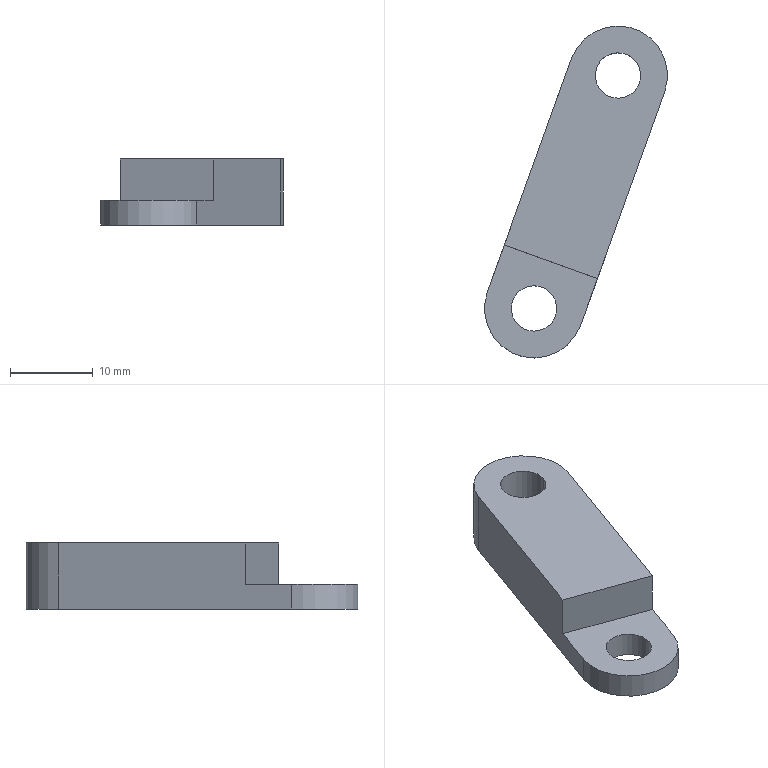Component | SolidWorks | CLS-MechanismAccessory3-1 | 1 solid | 12 faces | box 22.17 x 40.22 x 8 mm | volume 2881 mm3 | cylinder 6 | plane 6 | commonest cylinder face diameters 5.5 x4 12 x2
build123d program:
from build123d import *

# Parameters (mm, degrees)
SKETCH4_R           = 2.75
BOSS_EXTRUDE1_DEPTH = 8
SKETCH5_W           = 12
SKETCH5_H           = 24
CUT_EXTRUDE1_DEPTH  = 5


with BuildPart() as part:
    # Sketch4 → Boss-Extrude1 (new body)
    with BuildSketch(Plane.XY):
        with BuildLine():
            Line((6, 15), (6, -15))
            ThreePointArc((6, -15), (0, -21), (-6, -15))
            Line((-6, -15), (-6, 15))
            ThreePointArc((-6, 15), (0, 21), (6, 15))
        make_face()
        with Locations((0, 15)):
            Circle(SKETCH4_R, mode=Mode.SUBTRACT)
        with Locations((0, -15)):
            Circle(SKETCH4_R, mode=Mode.SUBTRACT)
    extrude(amount=BOSS_EXTRUDE1_DEPTH)

    # Sketch5 → Cut-Extrude1 (cut)
    with BuildSketch(Plane.XY):
        with Locations((0, -21)):
            Rectangle(SKETCH5_W, SKETCH5_H)
    extrude(amount=CUT_EXTRUDE1_DEPTH, mode=Mode.SUBTRACT)


solid = part.part

# Placed as in the assembly
solid = solid.moved(Location((58.557, -8.696, -5.001), (-180, 0, -160.191)))
STEP:
#1=COLOUR_RGB('',0.7922,0.8196,0.9333);
#2=FILL_AREA_STYLE_COLOUR('',#1);
#3=FILL_AREA_STYLE('',(#2));
#4=SURFACE_STYLE_FILL_AREA(#3);
#5=SURFACE_SIDE_STYLE('',(#4));
#6=SURFACE_STYLE_USAGE(.BOTH.,#5);
#7=PRESENTATION_STYLE_ASSIGNMENT((#6));
#8=CARTESIAN_POINT('',(2.607,0.1766,-0.5118));
#9=VERTEX_POINT('',#8);
#10=CARTESIAN_POINT('',(2.404,0.25,-0.5118));
#11=VERTEX_POINT('',#10);
#12=CARTESIAN_POINT('',(2.506,0.2133,-0.5118));
#13=DIRECTION('',(0.,0.,-1.));
#14=DIRECTION('',(-0.9408,0.3389,0.));
#15=AXIS2_PLACEMENT_3D('',#12,#13,#14);
#16=CIRCLE('',#15,0.1083);
#17=EDGE_CURVE('',#9,#11,#16,.T.);
#18=ORIENTED_EDGE('',*,*,#17,.T.);
#19=CARTESIAN_POINT('',(2.404,0.25,-0.1969));
#20=VERTEX_POINT('',#19);
#21=CARTESIAN_POINT('',(2.404,0.25,-0.5118));
#22=DIRECTION('',(-0.,-0.,1.));
#23=VECTOR('',#22,39.37);
#24=LINE('',#21,#23);
#25=EDGE_CURVE('',#11,#20,#24,.T.);
#26=ORIENTED_EDGE('',*,*,#25,.T.);
#27=CARTESIAN_POINT('',(2.607,0.1766,-0.1969));
#28=VERTEX_POINT('',#27);
#29=CARTESIAN_POINT('',(2.506,0.2133,-0.1969));
#30=DIRECTION('',(0.,0.,-1.));
#31=DIRECTION('',(-0.9408,0.3389,0.));
#32=AXIS2_PLACEMENT_3D('',#29,#30,#31);
#33=CIRCLE('',#32,0.1083);
#34=EDGE_CURVE('',#28,#20,#33,.T.);
#35=ORIENTED_EDGE('',*,*,#34,.F.);
#36=CARTESIAN_POINT('',(2.607,0.1766,-0.5118));
#37=DIRECTION('',(-0.,-0.,1.));
#38=VECTOR('',#37,39.37);
#39=LINE('',#36,#38);
#40=EDGE_CURVE('',#9,#28,#39,.T.);
#41=ORIENTED_EDGE('',*,*,#40,.F.);
#42=EDGE_LOOP('',(#18,#26,#35,#41));
#43=FACE_OUTER_BOUND('',#42,.T.);
#44=CARTESIAN_POINT('',(2.506,0.2133,-0.5118));
#45=DIRECTION('',(-0.,-0.,1.));
#46=DIRECTION('',(0.9408,-0.3389,0.));
#47=AXIS2_PLACEMENT_3D('',#44,#45,#46);
#48=CYLINDRICAL_SURFACE('',#47,0.1083);
#49=ADVANCED_FACE('',(#43),#48,.F.);
#50=CARTESIAN_POINT('',(2.207,-0.9346,-0.5118));
#51=VERTEX_POINT('',#50);
#52=CARTESIAN_POINT('',(2.003,-0.8613,-0.5118));
#53=VERTEX_POINT('',#52);
#54=CARTESIAN_POINT('',(2.105,-0.8979,-0.5118));
#55=DIRECTION('',(0.,0.,-1.));
#56=DIRECTION('',(-0.9408,0.3389,0.));
#57=AXIS2_PLACEMENT_3D('',#54,#55,#56);
#58=CIRCLE('',#57,0.1083);
#59=EDGE_CURVE('',#51,#53,#58,.T.);
#60=ORIENTED_EDGE('',*,*,#59,.T.);
#61=CARTESIAN_POINT('',(2.003,-0.8613,-0.3937));
#62=VERTEX_POINT('',#61);
#63=CARTESIAN_POINT('',(2.003,-0.8613,-0.5118));
#64=DIRECTION('',(-0.,-0.,1.));
#65=VECTOR('',#64,39.37);
#66=LINE('',#63,#65);
#67=EDGE_CURVE('',#53,#62,#66,.T.);
#68=ORIENTED_EDGE('',*,*,#67,.T.);
#69=CARTESIAN_POINT('',(2.207,-0.9346,-0.3937));
#70=VERTEX_POINT('',#69);
#71=CARTESIAN_POINT('',(2.105,-0.8979,-0.3937));
#72=DIRECTION('',(-0.,-0.,1.));
#73=DIRECTION('',(0.9408,-0.3389,0.));
#74=AXIS2_PLACEMENT_3D('',#71,#72,#73);
#75=CIRCLE('',#74,0.1083);
#76=EDGE_CURVE('',#62,#70,#75,.T.);
#77=ORIENTED_EDGE('',*,*,#76,.T.);
#78=CARTESIAN_POINT('',(2.207,-0.9346,-0.5118));
#79=DIRECTION('',(-0.,-0.,1.));
#80=VECTOR('',#79,39.37);
#81=LINE('',#78,#80);
#82=EDGE_CURVE('',#51,#70,#81,.T.);
#83=ORIENTED_EDGE('',*,*,#82,.F.);
#84=EDGE_LOOP('',(#60,#68,#77,#83));
#85=FACE_OUTER_BOUND('',#84,.T.);
#86=CARTESIAN_POINT('',(2.105,-0.8979,-0.5118));
#87=DIRECTION('',(-0.,-0.,1.));
#88=DIRECTION('',(0.9408,-0.3389,0.));
#89=AXIS2_PLACEMENT_3D('',#86,#87,#88);
#90=CYLINDRICAL_SURFACE('',#89,0.1083);
#91=ADVANCED_FACE('',(#85),#90,.F.);
#92=ORIENTED_EDGE('',*,*,#34,.T.);
#93=CARTESIAN_POINT('',(2.506,0.2133,-0.1969));
#94=DIRECTION('',(0.,0.,-1.));
#95=DIRECTION('',(-0.9408,0.3389,0.));
#96=AXIS2_PLACEMENT_3D('',#93,#94,#95);
#97=CIRCLE('',#96,0.1083);
#98=EDGE_CURVE('',#20,#28,#97,.T.);
#99=ORIENTED_EDGE('',*,*,#98,.T.);
#100=EDGE_LOOP('',(#92,#99));
#101=FACE_BOUND('',#100,.T.);
#102=CARTESIAN_POINT('',(1.963,-0.5957,-0.1969));
#103=VERTEX_POINT('',#102);
#104=CARTESIAN_POINT('',(2.408,-0.7558,-0.1969));
#105=VERTEX_POINT('',#104);
#106=CARTESIAN_POINT('',(2.408,-0.7558,-0.1969));
#107=DIRECTION('',(0.9408,-0.3389,-0.));
#108=VECTOR('',#107,39.37);
#109=LINE('',#106,#108);
#110=EDGE_CURVE('',#103,#105,#109,.T.);
#111=ORIENTED_EDGE('',*,*,#110,.T.);
#112=CARTESIAN_POINT('',(2.728,0.1332,-0.1969));
#113=VERTEX_POINT('',#112);
#114=CARTESIAN_POINT('',(2.728,0.1332,-0.1969));
#115=DIRECTION('',(-0.3389,-0.9408,-0.));
#116=VECTOR('',#115,39.37);
#117=LINE('',#114,#116);
#118=EDGE_CURVE('',#113,#105,#117,.T.);
#119=ORIENTED_EDGE('',*,*,#118,.F.);
#120=CARTESIAN_POINT('',(2.283,0.2933,-0.1969));
#121=VERTEX_POINT('',#120);
#122=CARTESIAN_POINT('',(2.506,0.2133,-0.1969));
#123=DIRECTION('',(0.,0.,-1.));
#124=DIRECTION('',(-0.9408,0.3389,0.));
#125=AXIS2_PLACEMENT_3D('',#122,#123,#124);
#126=CIRCLE('',#125,0.2362);
#127=EDGE_CURVE('',#121,#113,#126,.T.);
#128=ORIENTED_EDGE('',*,*,#127,.F.);
#129=CARTESIAN_POINT('',(2.283,0.2933,-0.1969));
#130=DIRECTION('',(0.3389,0.9408,0.));
#131=VECTOR('',#130,39.37);
#132=LINE('',#129,#131);
#133=EDGE_CURVE('',#103,#121,#132,.T.);
#134=ORIENTED_EDGE('',*,*,#133,.F.);
#135=EDGE_LOOP('',(#111,#119,#128,#134));
#136=FACE_OUTER_BOUND('',#135,.T.);
#137=CARTESIAN_POINT('',(2.506,0.2133,-0.1969));
#138=DIRECTION('',(0.,0.,-1.));
#139=DIRECTION('',(-0.9408,0.3389,0.));
#140=AXIS2_PLACEMENT_3D('',#137,#138,#139);
#141=PLANE('',#140);
#142=ADVANCED_FACE('',(#101,#136),#141,.F.);
#143=CARTESIAN_POINT('',(2.408,-0.7558,-0.3937));
#144=VERTEX_POINT('',#143);
#145=CARTESIAN_POINT('',(2.408,-0.7558,-0.3937));
#146=DIRECTION('',(-0.,-0.,1.));
#147=VECTOR('',#146,39.37);
#148=LINE('',#145,#147);
#149=EDGE_CURVE('',#144,#105,#148,.T.);
#150=ORIENTED_EDGE('',*,*,#149,.F.);
#151=CARTESIAN_POINT('',(2.328,-0.978,-0.3937));
#152=VERTEX_POINT('',#151);
#153=CARTESIAN_POINT('',(2.087,-1.645,-0.3937));
#154=DIRECTION('',(-0.3389,-0.9408,-0.));
#155=VECTOR('',#154,39.37);
#156=LINE('',#153,#155);
#157=EDGE_CURVE('',#144,#152,#156,.T.);
#158=ORIENTED_EDGE('',*,*,#157,.T.);
#159=CARTESIAN_POINT('',(2.328,-0.978,-0.5118));
#160=VERTEX_POINT('',#159);
#161=CARTESIAN_POINT('',(2.328,-0.978,-0.5118));
#162=DIRECTION('',(-0.,-0.,1.));
#163=VECTOR('',#162,39.37);
#164=LINE('',#161,#163);
#165=EDGE_CURVE('',#160,#152,#164,.T.);
#166=ORIENTED_EDGE('',*,*,#165,.F.);
#167=CARTESIAN_POINT('',(2.728,0.1332,-0.5118));
#168=VERTEX_POINT('',#167);
#169=CARTESIAN_POINT('',(2.728,0.1332,-0.5118));
#170=DIRECTION('',(-0.3389,-0.9408,-0.));
#171=VECTOR('',#170,39.37);
#172=LINE('',#169,#171);
#173=EDGE_CURVE('',#168,#160,#172,.T.);
#174=ORIENTED_EDGE('',*,*,#173,.F.);
#175=CARTESIAN_POINT('',(2.728,0.1332,-0.5118));
#176=DIRECTION('',(-0.,-0.,1.));
#177=VECTOR('',#176,39.37);
#178=LINE('',#175,#177);
#179=EDGE_CURVE('',#168,#113,#178,.T.);
#180=ORIENTED_EDGE('',*,*,#179,.T.);
#181=ORIENTED_EDGE('',*,*,#118,.T.);
#182=EDGE_LOOP('',(#150,#158,#166,#174,#180,#181));
#183=FACE_OUTER_BOUND('',#182,.T.);
#184=CARTESIAN_POINT('',(2.728,0.1332,-0.5118));
#185=DIRECTION('',(-0.9408,0.3389,0.));
#186=DIRECTION('',(-0.,-0.,1.));
#187=AXIS2_PLACEMENT_3D('',#184,#185,#186);
#188=PLANE('',#187);
#189=ADVANCED_FACE('',(#183),#188,.F.);
#190=CARTESIAN_POINT('',(1.883,-0.8179,-0.3937));
#191=VERTEX_POINT('',#190);
#192=CARTESIAN_POINT('',(2.105,-0.8979,-0.3937));
#193=DIRECTION('',(-0.,-0.,1.));
#194=DIRECTION('',(0.9408,-0.3389,0.));
#195=AXIS2_PLACEMENT_3D('',#192,#193,#194);
#196=CIRCLE('',#195,0.2362);
#197=EDGE_CURVE('',#191,#152,#196,.T.);
#198=ORIENTED_EDGE('',*,*,#197,.F.);
#199=CARTESIAN_POINT('',(1.883,-0.8179,-0.5118));
#200=VERTEX_POINT('',#199);
#201=CARTESIAN_POINT('',(1.883,-0.8179,-0.5118));
#202=DIRECTION('',(-0.,-0.,1.));
#203=VECTOR('',#202,39.37);
#204=LINE('',#201,#203);
#205=EDGE_CURVE('',#200,#191,#204,.T.);
#206=ORIENTED_EDGE('',*,*,#205,.F.);
#207=CARTESIAN_POINT('',(2.105,-0.8979,-0.5118));
#208=DIRECTION('',(0.,0.,-1.));
#209=DIRECTION('',(-0.9408,0.3389,0.));
#210=AXIS2_PLACEMENT_3D('',#207,#208,#209);
#211=CIRCLE('',#210,0.2362);
#212=EDGE_CURVE('',#160,#200,#211,.T.);
#213=ORIENTED_EDGE('',*,*,#212,.F.);
#214=ORIENTED_EDGE('',*,*,#165,.T.);
#215=EDGE_LOOP('',(#198,#206,#213,#214));
#216=FACE_OUTER_BOUND('',#215,.T.);
#217=CARTESIAN_POINT('',(2.105,-0.8979,-0.5118));
#218=DIRECTION('',(-0.,-0.,1.));
#219=DIRECTION('',(0.9408,-0.3389,0.));
#220=AXIS2_PLACEMENT_3D('',#217,#218,#219);
#221=CYLINDRICAL_SURFACE('',#220,0.2362);
#222=ADVANCED_FACE('',(#216),#221,.T.);
#223=CARTESIAN_POINT('',(1.963,-0.5957,-0.3937));
#224=VERTEX_POINT('',#223);
#225=CARTESIAN_POINT('',(1.963,-0.5957,-0.3937));
#226=DIRECTION('',(-0.,-0.,1.));
#227=VECTOR('',#226,39.37);
#228=LINE('',#225,#227);
#229=EDGE_CURVE('',#224,#103,#228,.T.);
#230=ORIENTED_EDGE('',*,*,#229,.T.);
#231=ORIENTED_EDGE('',*,*,#133,.T.);
#232=CARTESIAN_POINT('',(2.283,0.2933,-0.5118));
#233=VERTEX_POINT('',#232);
#234=CARTESIAN_POINT('',(2.283,0.2933,-0.5118));
#235=DIRECTION('',(-0.,-0.,1.));
#236=VECTOR('',#235,39.37);
#237=LINE('',#234,#236);
#238=EDGE_CURVE('',#233,#121,#237,.T.);
#239=ORIENTED_EDGE('',*,*,#238,.F.);
#240=CARTESIAN_POINT('',(2.283,0.2933,-0.5118));
#241=DIRECTION('',(0.3389,0.9408,0.));
#242=VECTOR('',#241,39.37);
#243=LINE('',#240,#242);
#244=EDGE_CURVE('',#200,#233,#243,.T.);
#245=ORIENTED_EDGE('',*,*,#244,.F.);
#246=ORIENTED_EDGE('',*,*,#205,.T.);
#247=CARTESIAN_POINT('',(1.643,-1.485,-0.3937));
#248=DIRECTION('',(0.3389,0.9408,0.));
#249=VECTOR('',#248,39.37);
#250=LINE('',#247,#249);
#251=EDGE_CURVE('',#191,#224,#250,.T.);
#252=ORIENTED_EDGE('',*,*,#251,.T.);
#253=EDGE_LOOP('',(#230,#231,#239,#245,#246,#252));
#254=FACE_OUTER_BOUND('',#253,.T.);
#255=CARTESIAN_POINT('',(2.283,0.2933,-0.5118));
#256=DIRECTION('',(0.9408,-0.3389,-0.));
#257=DIRECTION('',(-0.3389,-0.9408,-0.));
#258=AXIS2_PLACEMENT_3D('',#255,#256,#257);
#259=PLANE('',#258);
#260=ADVANCED_FACE('',(#254),#259,.F.);
#261=ORIENTED_EDGE('',*,*,#67,.F.);
#262=CARTESIAN_POINT('',(2.105,-0.8979,-0.5118));
#263=DIRECTION('',(0.,0.,-1.));
#264=DIRECTION('',(-0.9408,0.3389,0.));
#265=AXIS2_PLACEMENT_3D('',#262,#263,#264);
#266=CIRCLE('',#265,0.1083);
#267=EDGE_CURVE('',#53,#51,#266,.T.);
#268=ORIENTED_EDGE('',*,*,#267,.T.);
#269=ORIENTED_EDGE('',*,*,#82,.T.);
#270=CARTESIAN_POINT('',(2.105,-0.8979,-0.3937));
#271=DIRECTION('',(-0.,-0.,1.));
#272=DIRECTION('',(0.9408,-0.3389,0.));
#273=AXIS2_PLACEMENT_3D('',#270,#271,#272);
#274=CIRCLE('',#273,0.1083);
#275=EDGE_CURVE('',#70,#62,#274,.T.);
#276=ORIENTED_EDGE('',*,*,#275,.T.);
#277=EDGE_LOOP('',(#261,#268,#269,#276));
#278=FACE_OUTER_BOUND('',#277,.T.);
#279=CARTESIAN_POINT('',(2.105,-0.8979,-0.5118));
#280=DIRECTION('',(-0.,-0.,1.));
#281=DIRECTION('',(0.9408,-0.3389,0.));
#282=AXIS2_PLACEMENT_3D('',#279,#280,#281);
#283=CYLINDRICAL_SURFACE('',#282,0.1083);
#284=ADVANCED_FACE('',(#278),#283,.F.);
#285=ORIENTED_EDGE('',*,*,#17,.F.);
#286=CARTESIAN_POINT('',(2.506,0.2133,-0.5118));
#287=DIRECTION('',(0.,0.,-1.));
#288=DIRECTION('',(-0.9408,0.3389,0.));
#289=AXIS2_PLACEMENT_3D('',#286,#287,#288);
#290=CIRCLE('',#289,0.1083);
#291=EDGE_CURVE('',#11,#9,#290,.T.);
#292=ORIENTED_EDGE('',*,*,#291,.F.);
#293=EDGE_LOOP('',(#285,#292));
#294=FACE_BOUND('',#293,.T.);
#295=CARTESIAN_POINT('',(2.506,0.2133,-0.5118));
#296=DIRECTION('',(0.,0.,-1.));
#297=DIRECTION('',(-0.9408,0.3389,0.));
#298=AXIS2_PLACEMENT_3D('',#295,#296,#297);
#299=CIRCLE('',#298,0.2362);
#300=EDGE_CURVE('',#233,#168,#299,.T.);
#301=ORIENTED_EDGE('',*,*,#300,.T.);
#302=ORIENTED_EDGE('',*,*,#173,.T.);
#303=ORIENTED_EDGE('',*,*,#212,.T.);
#304=ORIENTED_EDGE('',*,*,#244,.T.);
#305=EDGE_LOOP('',(#301,#302,#303,#304));
#306=FACE_OUTER_BOUND('',#305,.T.);
#307=ORIENTED_EDGE('',*,*,#59,.F.);
#308=ORIENTED_EDGE('',*,*,#267,.F.);
#309=EDGE_LOOP('',(#307,#308));
#310=FACE_BOUND('',#309,.T.);
#311=CARTESIAN_POINT('',(2.506,0.2133,-0.5118));
#312=DIRECTION('',(0.,0.,-1.));
#313=DIRECTION('',(-0.9408,0.3389,0.));
#314=AXIS2_PLACEMENT_3D('',#311,#312,#313);
#315=PLANE('',#314);
#316=ADVANCED_FACE('',(#294,#306,#310),#315,.T.);
#317=ORIENTED_EDGE('',*,*,#127,.T.);
#318=ORIENTED_EDGE('',*,*,#179,.F.);
#319=ORIENTED_EDGE('',*,*,#300,.F.);
#320=ORIENTED_EDGE('',*,*,#238,.T.);
#321=EDGE_LOOP('',(#317,#318,#319,#320));
#322=FACE_OUTER_BOUND('',#321,.T.);
#323=CARTESIAN_POINT('',(2.506,0.2133,-0.5118));
#324=DIRECTION('',(-0.,-0.,1.));
#325=DIRECTION('',(0.9408,-0.3389,0.));
#326=AXIS2_PLACEMENT_3D('',#323,#324,#325);
#327=CYLINDRICAL_SURFACE('',#326,0.2362);
#328=ADVANCED_FACE('',(#322),#327,.T.);
#329=ORIENTED_EDGE('',*,*,#25,.F.);
#330=ORIENTED_EDGE('',*,*,#291,.T.);
#331=ORIENTED_EDGE('',*,*,#40,.T.);
#332=ORIENTED_EDGE('',*,*,#98,.F.);
#333=EDGE_LOOP('',(#329,#330,#331,#332));
#334=FACE_OUTER_BOUND('',#333,.T.);
#335=CARTESIAN_POINT('',(2.506,0.2133,-0.5118));
#336=DIRECTION('',(-0.,-0.,1.));
#337=DIRECTION('',(0.9408,-0.3389,0.));
#338=AXIS2_PLACEMENT_3D('',#335,#336,#337);
#339=CYLINDRICAL_SURFACE('',#338,0.1083);
#340=ADVANCED_FACE('',(#334),#339,.F.);
#341=ORIENTED_EDGE('',*,*,#275,.F.);
#342=ORIENTED_EDGE('',*,*,#76,.F.);
#343=EDGE_LOOP('',(#341,#342));
#344=FACE_BOUND('',#343,.T.);
#345=ORIENTED_EDGE('',*,*,#197,.T.);
#346=ORIENTED_EDGE('',*,*,#157,.F.);
#347=CARTESIAN_POINT('',(2.408,-0.7558,-0.3937));
#348=DIRECTION('',(0.9408,-0.3389,-0.));
#349=VECTOR('',#348,39.37);
#350=LINE('',#347,#349);
#351=EDGE_CURVE('',#224,#144,#350,.T.);
#352=ORIENTED_EDGE('',*,*,#351,.F.);
#353=ORIENTED_EDGE('',*,*,#251,.F.);
#354=EDGE_LOOP('',(#345,#346,#352,#353));
#355=FACE_OUTER_BOUND('',#354,.T.);
#356=CARTESIAN_POINT('',(1.963,-0.5957,-0.3937));
#357=DIRECTION('',(-0.,-0.,1.));
#358=DIRECTION('',(0.9408,-0.3389,-0.));
#359=AXIS2_PLACEMENT_3D('',#356,#357,#358);
#360=PLANE('',#359);
#361=ADVANCED_FACE('',(#344,#355),#360,.T.);
#362=ORIENTED_EDGE('',*,*,#110,.F.);
#363=ORIENTED_EDGE('',*,*,#229,.F.);
#364=ORIENTED_EDGE('',*,*,#351,.T.);
#365=ORIENTED_EDGE('',*,*,#149,.T.);
#366=EDGE_LOOP('',(#362,#363,#364,#365));
#367=FACE_OUTER_BOUND('',#366,.T.);
#368=CARTESIAN_POINT('',(2.408,-0.7558,-0.3937));
#369=DIRECTION('',(-0.3389,-0.9408,-0.));
#370=DIRECTION('',(-0.,-0.,1.));
#371=AXIS2_PLACEMENT_3D('',#368,#369,#370);
#372=PLANE('',#371);
#373=ADVANCED_FACE('',(#367),#372,.T.);
#374=CLOSED_SHELL('',(#49,#91,#142,#189,#222,#260,#284,#316,#328,#340,#361,#373));
#375=MANIFOLD_SOLID_BREP('',#374);
#376=STYLED_ITEM('',(#7),#375);
#377=(LENGTH_UNIT()NAMED_UNIT(*)SI_UNIT($,.METRE.));
#378=LENGTH_MEASURE_WITH_UNIT(LENGTH_MEASURE(0.0254),#377);
#379=DIMENSIONAL_EXPONENTS(1.,0.,0.,0.,0.,0.,0.);
#380=(CONVERSION_BASED_UNIT('',#378)LENGTH_UNIT()NAMED_UNIT(#379));
#381=UNCERTAINTY_MEASURE_WITH_UNIT(LENGTH_MEASURE(0.00001),#380,'','');
#382=(NAMED_UNIT(*)PLANE_ANGLE_UNIT()SI_UNIT($,.RADIAN.));
#383=(NAMED_UNIT(*)SI_UNIT($,.STERADIAN.)SOLID_ANGLE_UNIT());
#384=(GEOMETRIC_REPRESENTATION_CONTEXT(3)GLOBAL_UNCERTAINTY_ASSIGNED_CONTEXT((#381))GLOBAL_UNIT_ASSIGNED_CONTEXT((#380,#382,#383))REPRESENTATION_CONTEXT('',''));
#385=MECHANICAL_DESIGN_GEOMETRIC_PRESENTATION_REPRESENTATION('',(#376),#384);
#386=PRESENTATION_LAYER_ASSIGNMENT('','',(#376));
#387=CARTESIAN_POINT('',(0.,0.,0.));
#388=DIRECTION('',(0.,0.,1.));
#389=DIRECTION('',(1.,0.,0.));
#390=AXIS2_PLACEMENT_3D('',#387,#388,#389);
#391=(LENGTH_UNIT()NAMED_UNIT(*)SI_UNIT($,.METRE.));
#392=LENGTH_MEASURE_WITH_UNIT(LENGTH_MEASURE(0.0254),#391);
#393=DIMENSIONAL_EXPONENTS(1.,0.,0.,0.,0.,0.,0.);
#394=(CONVERSION_BASED_UNIT('',#392)LENGTH_UNIT()NAMED_UNIT(#393));
#395=UNCERTAINTY_MEASURE_WITH_UNIT(LENGTH_MEASURE(0.00001),#394,'','');
#396=(NAMED_UNIT(*)PLANE_ANGLE_UNIT()SI_UNIT($,.RADIAN.));
#397=(NAMED_UNIT(*)SI_UNIT($,.STERADIAN.)SOLID_ANGLE_UNIT());
#398=(GEOMETRIC_REPRESENTATION_CONTEXT(3)GLOBAL_UNCERTAINTY_ASSIGNED_CONTEXT((#395))GLOBAL_UNIT_ASSIGNED_CONTEXT((#394,#396,#397))REPRESENTATION_CONTEXT('',''));
#399=ADVANCED_BREP_SHAPE_REPRESENTATION('',(#375,#390),#398);